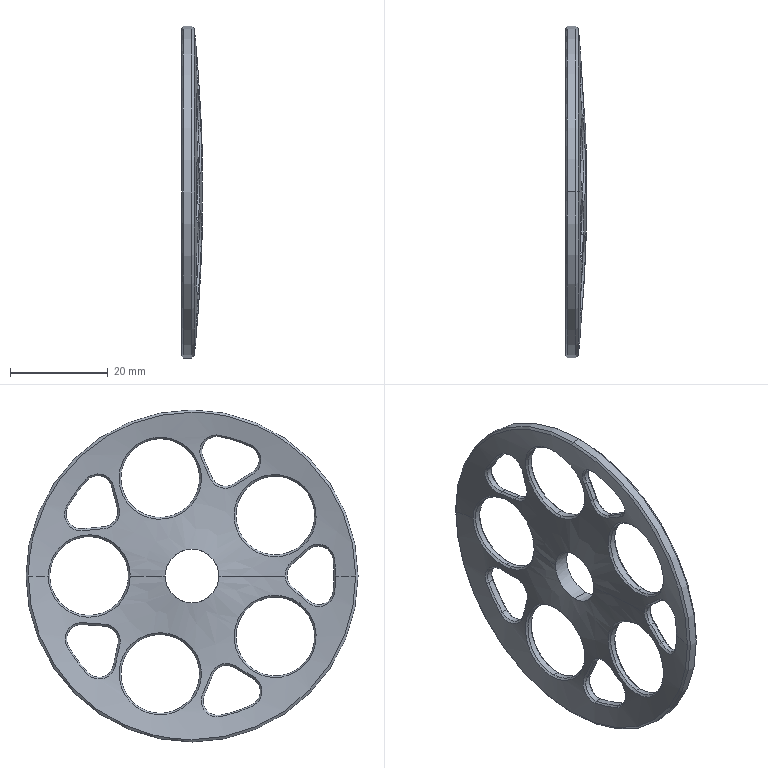CAM job | Mastercam | mm | 3 operations | part box 4.24 x 67.9 x 67.9
1. Lathe Rough | 1 - OD ROUGH RIGHT - 80 DEG.
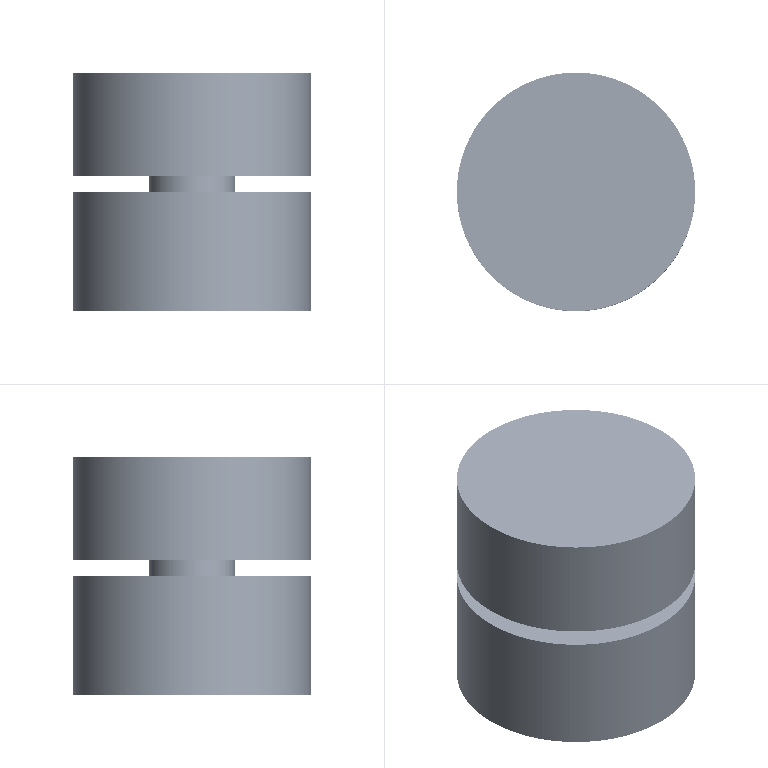2. C-Axis Face Contour | 2 - 6 平铣刀
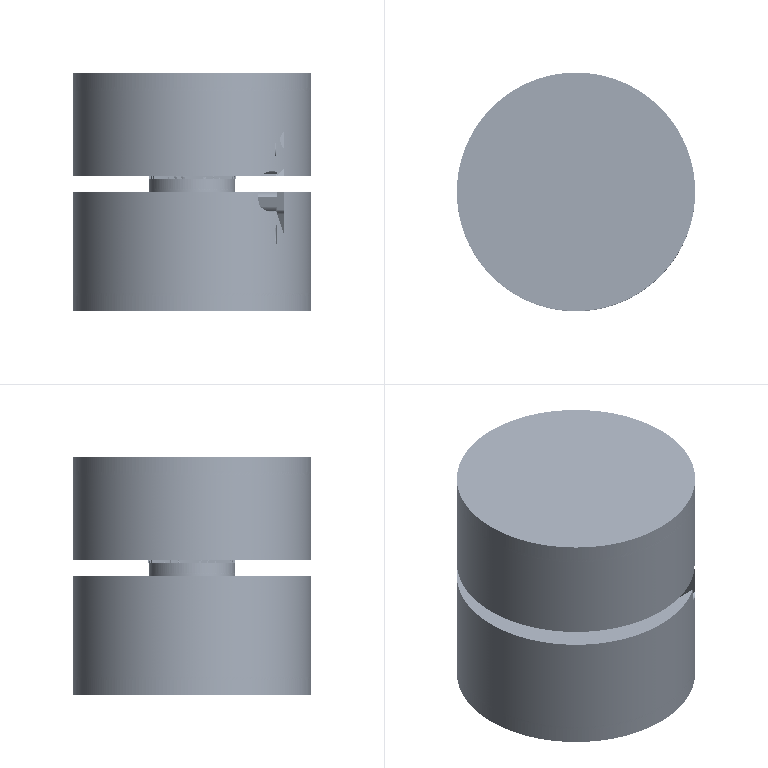3. C-Axis Face Contour | 3 - 6 倒角铣刀